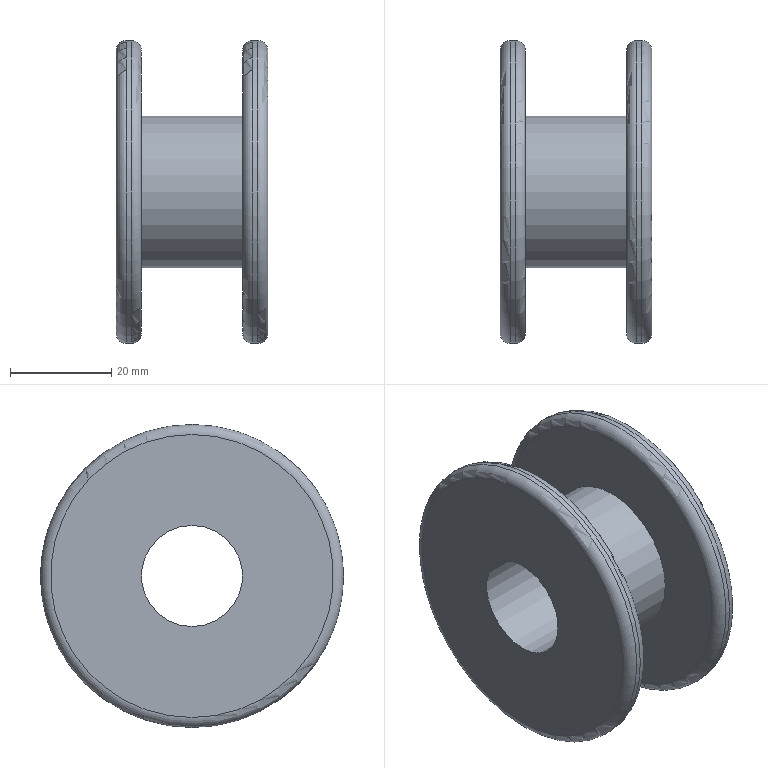Component | NX | 2 | 1 solid | 12 faces | box 30 x 60 x 60 mm | volume 32349 mm3 | cylinder 4 | plane 4 | torus 4 | commonest cylinder face diameters 60 x2 30 x1 20 x1
STEP:
#1=CARTESIAN_POINT('',(0.,0.,0.));
#2=DIRECTION('',(0.,0.,1.));
#3=DIRECTION('',(1.,0.,0.));
#4=AXIS2_PLACEMENT_3D('',#1,#2,#3);
#5=CARTESIAN_POINT('',(10.,0.,23.));
#6=VERTEX_POINT('',#5);
#7=CARTESIAN_POINT('',(10.,0.,38.));
#8=DIRECTION('',(1.,0.,0.));
#9=DIRECTION('',(0.,0.,-1.));
#10=AXIS2_PLACEMENT_3D('',#7,#8,#9);
#11=CIRCLE('',#10,15.);
#12=CARTESIAN_POINT('',(-15.,0.,38.));
#13=DIRECTION('',(1.,0.,0.));
#14=DIRECTION('',(0.,-1.,0.));
#15=AXIS2_PLACEMENT_3D('',#12,#13,#14);
#16=CYLINDRICAL_SURFACE('',#15,15.);
#17=CARTESIAN_POINT('',(1.571,25.));
#18=DIRECTION('',(1.,0.));
#19=VECTOR('',#18,1.);
#20=LINE('',#17,#19);
#21=(GEOMETRIC_REPRESENTATION_CONTEXT(2)PARAMETRIC_REPRESENTATION_CONTEXT()REPRESENTATION_CONTEXT('',''));
#22=DEFINITIONAL_REPRESENTATION('',(#20),#21);
#23=PCURVE('',#16,#22);
#24=CARTESIAN_POINT('',(10.,0.,38.));
#25=DIRECTION('',(-1.,0.,0.));
#26=DIRECTION('',(0.,0.,-1.));
#27=AXIS2_PLACEMENT_3D('',#24,#25,#26);
#28=PLANE('',#27);
#29=CARTESIAN_POINT('',(15.,0.));
#30=CARTESIAN_POINT('',(15.,-25.981));
#31=CARTESIAN_POINT('',(-7.5,-12.99));
#32=CARTESIAN_POINT('',(-30.,-0.));
#33=CARTESIAN_POINT('',(-7.5,12.99));
#34=CARTESIAN_POINT('',(15.,25.981));
#35=CARTESIAN_POINT('',(15.,0.));
#36=(BOUNDED_CURVE()B_SPLINE_CURVE(2,(#29,#30,#31,#32,#33,#34,#35),.UNSPECIFIED.,.T.,.F.)B_SPLINE_CURVE_WITH_KNOTS((1,2,2,2,2,1),(-2.094,0.,2.094,4.189,6.283,8.378),.UNSPECIFIED.)CURVE()GEOMETRIC_REPRESENTATION_ITEM()RATIONAL_B_SPLINE_CURVE((1.,0.5,1.,0.5,1.,0.5,1.))REPRESENTATION_ITEM(''));
#37=(GEOMETRIC_REPRESENTATION_CONTEXT(2)PARAMETRIC_REPRESENTATION_CONTEXT()REPRESENTATION_CONTEXT('',''));
#38=DEFINITIONAL_REPRESENTATION('',(#36),#37);
#39=PCURVE('',#28,#38);
#40=SURFACE_CURVE('',#11,(#23,#39),.PCURVE_S1.);
#41=EDGE_CURVE('',#6,#6,#40,.T.);
#42=ORIENTED_EDGE('',*,*,#41,.F.);
#43=CARTESIAN_POINT('',(-10.,-0.,23.));
#44=VERTEX_POINT('',#43);
#45=CARTESIAN_POINT('',(-10.,-0.,23.));
#46=CARTESIAN_POINT('',(10.,-0.,23.));
#47=B_SPLINE_CURVE_WITH_KNOTS('',1,(#45,#46),.UNSPECIFIED.,.F.,.F.,(2,2),(5.,25.),.PIECEWISE_BEZIER_KNOTS.);
#48=CARTESIAN_POINT('',(1.571,0.));
#49=DIRECTION('',(0.,1.));
#50=VECTOR('',#49,1.);
#51=LINE('',#48,#50);
#52=(GEOMETRIC_REPRESENTATION_CONTEXT(2)PARAMETRIC_REPRESENTATION_CONTEXT()REPRESENTATION_CONTEXT('',''));
#53=DEFINITIONAL_REPRESENTATION('',(#51),#52);
#54=PCURVE('',#16,#53);
#55=CARTESIAN_POINT('',(7.854,0.));
#56=DIRECTION('',(0.,1.));
#57=VECTOR('',#56,1.);
#58=LINE('',#55,#57);
#59=(GEOMETRIC_REPRESENTATION_CONTEXT(2)PARAMETRIC_REPRESENTATION_CONTEXT()REPRESENTATION_CONTEXT('',''));
#60=DEFINITIONAL_REPRESENTATION('',(#58),#59);
#61=PCURVE('',#16,#60);
#62=SEAM_CURVE('',#47,(#54,#61),.PCURVE_S1.);
#63=EDGE_CURVE('',#44,#6,#62,.T.);
#64=ORIENTED_EDGE('',*,*,#63,.F.);
#65=CARTESIAN_POINT('',(-10.,0.,53.));
#66=VERTEX_POINT('',#65);
#67=CARTESIAN_POINT('',(-10.,0.,38.));
#68=DIRECTION('',(-1.,0.,0.));
#69=DIRECTION('',(0.,0.,1.));
#70=AXIS2_PLACEMENT_3D('',#67,#68,#69);
#71=CIRCLE('',#70,15.);
#72=CARTESIAN_POINT('',(4.712,5.));
#73=DIRECTION('',(-1.,0.));
#74=VECTOR('',#73,1.);
#75=LINE('',#72,#74);
#76=(GEOMETRIC_REPRESENTATION_CONTEXT(2)PARAMETRIC_REPRESENTATION_CONTEXT()REPRESENTATION_CONTEXT('',''));
#77=DEFINITIONAL_REPRESENTATION('',(#75),#76);
#78=PCURVE('',#16,#77);
#79=CARTESIAN_POINT('',(-10.,0.,38.));
#80=DIRECTION('',(1.,0.,0.));
#81=DIRECTION('',(0.,0.,1.));
#82=AXIS2_PLACEMENT_3D('',#79,#80,#81);
#83=PLANE('',#82);
#84=CARTESIAN_POINT('',(15.,0.));
#85=CARTESIAN_POINT('',(15.,-25.981));
#86=CARTESIAN_POINT('',(-7.5,-12.99));
#87=CARTESIAN_POINT('',(-30.,-0.));
#88=CARTESIAN_POINT('',(-7.5,12.99));
#89=CARTESIAN_POINT('',(15.,25.981));
#90=CARTESIAN_POINT('',(15.,0.));
#91=(BOUNDED_CURVE()B_SPLINE_CURVE(2,(#84,#85,#86,#87,#88,#89,#90),.UNSPECIFIED.,.T.,.F.)B_SPLINE_CURVE_WITH_KNOTS((1,2,2,2,2,1),(-2.094,0.,2.094,4.189,6.283,8.378),.UNSPECIFIED.)CURVE()GEOMETRIC_REPRESENTATION_ITEM()RATIONAL_B_SPLINE_CURVE((1.,0.5,1.,0.5,1.,0.5,1.))REPRESENTATION_ITEM(''));
#92=(GEOMETRIC_REPRESENTATION_CONTEXT(2)PARAMETRIC_REPRESENTATION_CONTEXT()REPRESENTATION_CONTEXT('',''));
#93=DEFINITIONAL_REPRESENTATION('',(#91),#92);
#94=PCURVE('',#83,#93);
#95=SURFACE_CURVE('',#71,(#78,#94),.PCURVE_S1.);
#96=EDGE_CURVE('',#66,#44,#95,.T.);
#97=ORIENTED_EDGE('',*,*,#96,.F.);
#98=CARTESIAN_POINT('',(-10.,0.,38.));
#99=DIRECTION('',(-1.,0.,0.));
#100=DIRECTION('',(0.,0.,1.));
#101=AXIS2_PLACEMENT_3D('',#98,#99,#100);
#102=CIRCLE('',#101,15.);
#103=CARTESIAN_POINT('',(10.996,5.));
#104=DIRECTION('',(-1.,0.));
#105=VECTOR('',#104,1.);
#106=LINE('',#103,#105);
#107=(GEOMETRIC_REPRESENTATION_CONTEXT(2)PARAMETRIC_REPRESENTATION_CONTEXT()REPRESENTATION_CONTEXT('',''));
#108=DEFINITIONAL_REPRESENTATION('',(#106),#107);
#109=PCURVE('',#16,#108);
#110=CARTESIAN_POINT('',(15.,0.));
#111=CARTESIAN_POINT('',(15.,-25.981));
#112=CARTESIAN_POINT('',(-7.5,-12.99));
#113=CARTESIAN_POINT('',(-30.,-0.));
#114=CARTESIAN_POINT('',(-7.5,12.99));
#115=CARTESIAN_POINT('',(15.,25.981));
#116=CARTESIAN_POINT('',(15.,0.));
#117=(BOUNDED_CURVE()B_SPLINE_CURVE(2,(#110,#111,#112,#113,#114,#115,#116),.UNSPECIFIED.,.T.,.F.)B_SPLINE_CURVE_WITH_KNOTS((1,2,2,2,2,1),(-2.094,0.,2.094,4.189,6.283,8.378),.UNSPECIFIED.)CURVE()GEOMETRIC_REPRESENTATION_ITEM()RATIONAL_B_SPLINE_CURVE((1.,0.5,1.,0.5,1.,0.5,1.))REPRESENTATION_ITEM(''));
#118=(GEOMETRIC_REPRESENTATION_CONTEXT(2)PARAMETRIC_REPRESENTATION_CONTEXT()REPRESENTATION_CONTEXT('',''));
#119=DEFINITIONAL_REPRESENTATION('',(#117),#118);
#120=PCURVE('',#83,#119);
#121=SURFACE_CURVE('',#102,(#109,#120),.PCURVE_S1.);
#122=EDGE_CURVE('',#44,#66,#121,.T.);
#123=ORIENTED_EDGE('',*,*,#122,.F.);
#124=ORIENTED_EDGE('',*,*,#63,.T.);
#125=EDGE_LOOP('',(#42,#64,#97,#123,#124));
#126=FACE_BOUND('',#125,.T.);
#127=ADVANCED_FACE('',(#126),#16,.T.);
#128=CARTESIAN_POINT('',(-10.,0.,66.));
#129=VERTEX_POINT('',#128);
#130=CARTESIAN_POINT('',(-10.,0.,38.));
#131=DIRECTION('',(1.,0.,0.));
#132=DIRECTION('',(0.,0.,1.));
#133=AXIS2_PLACEMENT_3D('',#130,#131,#132);
#134=CIRCLE('',#133,28.);
#135=CARTESIAN_POINT('',(0.,0.));
#136=DIRECTION('',(1.,0.));
#137=AXIS2_PLACEMENT_2D('',#135,#136);
#138=CIRCLE('',#137,28.);
#139=(GEOMETRIC_REPRESENTATION_CONTEXT(2)PARAMETRIC_REPRESENTATION_CONTEXT()REPRESENTATION_CONTEXT('',''));
#140=DEFINITIONAL_REPRESENTATION('',(#138),#139);
#141=PCURVE('',#83,#140);
#142=CARTESIAN_POINT('',(-12.,0.,38.));
#143=DIRECTION('',(1.,0.,0.));
#144=DIRECTION('',(0.,0.,1.));
#145=AXIS2_PLACEMENT_3D('',#142,#143,#144);
#146=TOROIDAL_SURFACE('',#145,28.,2.);
#147=CARTESIAN_POINT('',(0.,7.854));
#148=DIRECTION('',(1.,0.));
#149=VECTOR('',#148,1.);
#150=LINE('',#147,#149);
#151=(GEOMETRIC_REPRESENTATION_CONTEXT(2)PARAMETRIC_REPRESENTATION_CONTEXT()REPRESENTATION_CONTEXT('',''));
#152=DEFINITIONAL_REPRESENTATION('',(#150),#151);
#153=PCURVE('',#146,#152);
#154=SURFACE_CURVE('',#134,(#141,#153),.PCURVE_S1.);
#155=EDGE_CURVE('',#129,#129,#154,.T.);
#156=ORIENTED_EDGE('',*,*,#155,.T.);
#157=EDGE_LOOP('',(#156));
#158=FACE_BOUND('',#157,.T.);
#159=ORIENTED_EDGE('',*,*,#96,.T.);
#160=ORIENTED_EDGE('',*,*,#122,.T.);
#161=EDGE_LOOP('',(#159,#160));
#162=FACE_BOUND('',#161,.T.);
#163=ADVANCED_FACE('',(#158,#162),#83,.T.);
#164=CARTESIAN_POINT('',(-12.,0.,68.));
#165=VERTEX_POINT('',#164);
#166=CARTESIAN_POINT('',(-12.,0.,38.));
#167=DIRECTION('',(-1.,0.,0.));
#168=DIRECTION('',(0.,0.,1.));
#169=AXIS2_PLACEMENT_3D('',#166,#167,#168);
#170=CIRCLE('',#169,30.);
#171=CARTESIAN_POINT('',(-15.,0.,38.));
#172=DIRECTION('',(1.,0.,0.));
#173=DIRECTION('',(0.,-1.,0.));
#174=AXIS2_PLACEMENT_3D('',#171,#172,#173);
#175=CYLINDRICAL_SURFACE('',#174,30.);
#176=CARTESIAN_POINT('',(10.996,3.));
#177=DIRECTION('',(-1.,0.));
#178=VECTOR('',#177,1.);
#179=LINE('',#176,#178);
#180=(GEOMETRIC_REPRESENTATION_CONTEXT(2)PARAMETRIC_REPRESENTATION_CONTEXT()REPRESENTATION_CONTEXT('',''));
#181=DEFINITIONAL_REPRESENTATION('',(#179),#180);
#182=PCURVE('',#175,#181);
#183=CARTESIAN_POINT('',(6.283,6.283));
#184=DIRECTION('',(-1.,0.));
#185=VECTOR('',#184,1.);
#186=LINE('',#183,#185);
#187=(GEOMETRIC_REPRESENTATION_CONTEXT(2)PARAMETRIC_REPRESENTATION_CONTEXT()REPRESENTATION_CONTEXT('',''));
#188=DEFINITIONAL_REPRESENTATION('',(#186),#187);
#189=PCURVE('',#146,#188);
#190=SURFACE_CURVE('',#170,(#182,#189),.PCURVE_S1.);
#191=EDGE_CURVE('',#165,#165,#190,.T.);
#192=ORIENTED_EDGE('',*,*,#191,.T.);
#193=CARTESIAN_POINT('',(-13.,0.,68.));
#194=VERTEX_POINT('',#193);
#195=CARTESIAN_POINT('',(-13.,0.,68.));
#196=CARTESIAN_POINT('',(-12.,0.,68.));
#197=B_SPLINE_CURVE_WITH_KNOTS('',1,(#195,#196),.UNSPECIFIED.,.F.,.F.,(2,2),(2.,3.),.PIECEWISE_BEZIER_KNOTS.);
#198=CARTESIAN_POINT('',(4.712,0.));
#199=DIRECTION('',(0.,1.));
#200=VECTOR('',#199,1.);
#201=LINE('',#198,#200);
#202=(GEOMETRIC_REPRESENTATION_CONTEXT(2)PARAMETRIC_REPRESENTATION_CONTEXT()REPRESENTATION_CONTEXT('',''));
#203=DEFINITIONAL_REPRESENTATION('',(#201),#202);
#204=PCURVE('',#175,#203);
#205=CARTESIAN_POINT('',(10.996,0.));
#206=DIRECTION('',(0.,1.));
#207=VECTOR('',#206,1.);
#208=LINE('',#205,#207);
#209=(GEOMETRIC_REPRESENTATION_CONTEXT(2)PARAMETRIC_REPRESENTATION_CONTEXT()REPRESENTATION_CONTEXT('',''));
#210=DEFINITIONAL_REPRESENTATION('',(#208),#209);
#211=PCURVE('',#175,#210);
#212=SEAM_CURVE('',#197,(#204,#211),.PCURVE_S1.);
#213=EDGE_CURVE('',#194,#165,#212,.T.);
#214=ORIENTED_EDGE('',*,*,#213,.F.);
#215=CARTESIAN_POINT('',(-13.,0.,8.));
#216=VERTEX_POINT('',#215);
#217=CARTESIAN_POINT('',(-13.,0.,38.));
#218=DIRECTION('',(1.,0.,0.));
#219=DIRECTION('',(0.,0.,-1.));
#220=AXIS2_PLACEMENT_3D('',#217,#218,#219);
#221=CIRCLE('',#220,30.);
#222=CARTESIAN_POINT('',(1.571,2.));
#223=DIRECTION('',(1.,0.));
#224=VECTOR('',#223,1.);
#225=LINE('',#222,#224);
#226=(GEOMETRIC_REPRESENTATION_CONTEXT(2)PARAMETRIC_REPRESENTATION_CONTEXT()REPRESENTATION_CONTEXT('',''));
#227=DEFINITIONAL_REPRESENTATION('',(#225),#226);
#228=PCURVE('',#175,#227);
#229=CARTESIAN_POINT('',(-13.,0.,38.));
#230=DIRECTION('',(-1.,0.,0.));
#231=DIRECTION('',(0.,0.,-1.));
#232=AXIS2_PLACEMENT_3D('',#229,#230,#231);
#233=TOROIDAL_SURFACE('',#232,28.,2.);
#234=CARTESIAN_POINT('',(6.283,6.283));
#235=DIRECTION('',(-1.,0.));
#236=VECTOR('',#235,1.);
#237=LINE('',#234,#236);
#238=(GEOMETRIC_REPRESENTATION_CONTEXT(2)PARAMETRIC_REPRESENTATION_CONTEXT()REPRESENTATION_CONTEXT('',''));
#239=DEFINITIONAL_REPRESENTATION('',(#237),#238);
#240=PCURVE('',#233,#239);
#241=SURFACE_CURVE('',#221,(#228,#240),.PCURVE_S1.);
#242=EDGE_CURVE('',#194,#216,#241,.T.);
#243=ORIENTED_EDGE('',*,*,#242,.T.);
#244=CARTESIAN_POINT('',(-13.,0.,38.));
#245=DIRECTION('',(1.,0.,0.));
#246=DIRECTION('',(0.,0.,-1.));
#247=AXIS2_PLACEMENT_3D('',#244,#245,#246);
#248=CIRCLE('',#247,30.);
#249=CARTESIAN_POINT('',(7.854,2.));
#250=DIRECTION('',(1.,0.));
#251=VECTOR('',#250,1.);
#252=LINE('',#249,#251);
#253=(GEOMETRIC_REPRESENTATION_CONTEXT(2)PARAMETRIC_REPRESENTATION_CONTEXT()REPRESENTATION_CONTEXT('',''));
#254=DEFINITIONAL_REPRESENTATION('',(#252),#253);
#255=PCURVE('',#175,#254);
#256=CARTESIAN_POINT('',(6.283,6.283));
#257=DIRECTION('',(-1.,0.));
#258=VECTOR('',#257,1.);
#259=LINE('',#256,#258);
#260=(GEOMETRIC_REPRESENTATION_CONTEXT(2)PARAMETRIC_REPRESENTATION_CONTEXT()REPRESENTATION_CONTEXT('',''));
#261=DEFINITIONAL_REPRESENTATION('',(#259),#260);
#262=PCURVE('',#233,#261);
#263=SURFACE_CURVE('',#248,(#255,#262),.PCURVE_S1.);
#264=EDGE_CURVE('',#216,#194,#263,.T.);
#265=ORIENTED_EDGE('',*,*,#264,.T.);
#266=ORIENTED_EDGE('',*,*,#213,.T.);
#267=EDGE_LOOP('',(#192,#214,#243,#265,#266));
#268=FACE_BOUND('',#267,.T.);
#269=ADVANCED_FACE('',(#268),#175,.T.);
#270=CARTESIAN_POINT('',(-15.,0.,10.));
#271=VERTEX_POINT('',#270);
#272=CARTESIAN_POINT('',(-15.,0.,38.));
#273=DIRECTION('',(-1.,0.,0.));
#274=DIRECTION('',(0.,0.,-1.));
#275=AXIS2_PLACEMENT_3D('',#272,#273,#274);
#276=CIRCLE('',#275,28.);
#277=CARTESIAN_POINT('',(-15.,0.,38.));
#278=DIRECTION('',(-1.,0.,0.));
#279=DIRECTION('',(0.,0.,-1.));
#280=AXIS2_PLACEMENT_3D('',#277,#278,#279);
#281=PLANE('',#280);
#282=CARTESIAN_POINT('',(0.,0.));
#283=DIRECTION('',(1.,0.));
#284=AXIS2_PLACEMENT_2D('',#282,#283);
#285=CIRCLE('',#284,28.);
#286=(GEOMETRIC_REPRESENTATION_CONTEXT(2)PARAMETRIC_REPRESENTATION_CONTEXT()REPRESENTATION_CONTEXT('',''));
#287=DEFINITIONAL_REPRESENTATION('',(#285),#286);
#288=PCURVE('',#281,#287);
#289=CARTESIAN_POINT('',(0.,7.854));
#290=DIRECTION('',(1.,0.));
#291=VECTOR('',#290,1.);
#292=LINE('',#289,#291);
#293=(GEOMETRIC_REPRESENTATION_CONTEXT(2)PARAMETRIC_REPRESENTATION_CONTEXT()REPRESENTATION_CONTEXT('',''));
#294=DEFINITIONAL_REPRESENTATION('',(#292),#293);
#295=PCURVE('',#233,#294);
#296=SURFACE_CURVE('',#276,(#288,#295),.PCURVE_S1.);
#297=EDGE_CURVE('',#271,#271,#296,.T.);
#298=ORIENTED_EDGE('',*,*,#297,.T.);
#299=EDGE_LOOP('',(#298));
#300=FACE_BOUND('',#299,.T.);
#301=CARTESIAN_POINT('',(-15.,0.,48.));
#302=VERTEX_POINT('',#301);
#303=CARTESIAN_POINT('',(-15.,0.,38.));
#304=DIRECTION('',(1.,0.,0.));
#305=DIRECTION('',(0.,0.,1.));
#306=AXIS2_PLACEMENT_3D('',#303,#304,#305);
#307=CIRCLE('',#306,10.);
#308=CARTESIAN_POINT('',(-10.,0.));
#309=CARTESIAN_POINT('',(-10.,17.321));
#310=CARTESIAN_POINT('',(5.,8.66));
#311=CARTESIAN_POINT('',(20.,0.));
#312=CARTESIAN_POINT('',(5.,-8.66));
#313=CARTESIAN_POINT('',(-10.,-17.321));
#314=CARTESIAN_POINT('',(-10.,0.));
#315=(BOUNDED_CURVE()B_SPLINE_CURVE(2,(#308,#309,#310,#311,#312,#313,#314),.UNSPECIFIED.,.T.,.F.)B_SPLINE_CURVE_WITH_KNOTS((1,2,2,2,2,1),(-2.094,0.,2.094,4.189,6.283,8.378),.UNSPECIFIED.)CURVE()GEOMETRIC_REPRESENTATION_ITEM()RATIONAL_B_SPLINE_CURVE((1.,0.5,1.,0.5,1.,0.5,1.))REPRESENTATION_ITEM(''));
#316=(GEOMETRIC_REPRESENTATION_CONTEXT(2)PARAMETRIC_REPRESENTATION_CONTEXT()REPRESENTATION_CONTEXT('',''));
#317=DEFINITIONAL_REPRESENTATION('',(#315),#316);
#318=PCURVE('',#281,#317);
#319=CARTESIAN_POINT('',(-15.,0.,38.));
#320=DIRECTION('',(1.,0.,0.));
#321=DIRECTION('',(0.,0.,1.));
#322=AXIS2_PLACEMENT_3D('',#319,#320,#321);
#323=CYLINDRICAL_SURFACE('',#322,10.);
#324=CARTESIAN_POINT('',(0.,0.));
#325=DIRECTION('',(1.,0.));
#326=VECTOR('',#325,1.);
#327=LINE('',#324,#326);
#328=(GEOMETRIC_REPRESENTATION_CONTEXT(2)PARAMETRIC_REPRESENTATION_CONTEXT()REPRESENTATION_CONTEXT('',''));
#329=DEFINITIONAL_REPRESENTATION('',(#327),#328);
#330=PCURVE('',#323,#329);
#331=SURFACE_CURVE('',#307,(#318,#330),.PCURVE_S1.);
#332=EDGE_CURVE('',#302,#302,#331,.T.);
#333=ORIENTED_EDGE('',*,*,#332,.T.);
#334=EDGE_LOOP('',(#333));
#335=FACE_BOUND('',#334,.T.);
#336=ADVANCED_FACE('',(#300,#335),#281,.T.);
#337=CARTESIAN_POINT('',(10.,0.,10.));
#338=VERTEX_POINT('',#337);
#339=CARTESIAN_POINT('',(10.,0.,38.));
#340=DIRECTION('',(-1.,0.,0.));
#341=DIRECTION('',(0.,0.,-1.));
#342=AXIS2_PLACEMENT_3D('',#339,#340,#341);
#343=CIRCLE('',#342,28.);
#344=CARTESIAN_POINT('',(0.,0.));
#345=DIRECTION('',(1.,0.));
#346=AXIS2_PLACEMENT_2D('',#344,#345);
#347=CIRCLE('',#346,28.);
#348=(GEOMETRIC_REPRESENTATION_CONTEXT(2)PARAMETRIC_REPRESENTATION_CONTEXT()REPRESENTATION_CONTEXT('',''));
#349=DEFINITIONAL_REPRESENTATION('',(#347),#348);
#350=PCURVE('',#28,#349);
#351=CARTESIAN_POINT('',(12.,0.,38.));
#352=DIRECTION('',(-1.,0.,0.));
#353=DIRECTION('',(0.,0.,-1.));
#354=AXIS2_PLACEMENT_3D('',#351,#352,#353);
#355=TOROIDAL_SURFACE('',#354,28.,2.);
#356=CARTESIAN_POINT('',(0.,7.854));
#357=DIRECTION('',(1.,0.));
#358=VECTOR('',#357,1.);
#359=LINE('',#356,#358);
#360=(GEOMETRIC_REPRESENTATION_CONTEXT(2)PARAMETRIC_REPRESENTATION_CONTEXT()REPRESENTATION_CONTEXT('',''));
#361=DEFINITIONAL_REPRESENTATION('',(#359),#360);
#362=PCURVE('',#355,#361);
#363=SURFACE_CURVE('',#343,(#350,#362),.PCURVE_S1.);
#364=EDGE_CURVE('',#338,#338,#363,.T.);
#365=ORIENTED_EDGE('',*,*,#364,.T.);
#366=EDGE_LOOP('',(#365));
#367=FACE_BOUND('',#366,.T.);
#368=ORIENTED_EDGE('',*,*,#41,.T.);
#369=EDGE_LOOP('',(#368));
#370=FACE_BOUND('',#369,.T.);
#371=ADVANCED_FACE('',(#367,#370),#28,.T.);
#372=CARTESIAN_POINT('',(13.,0.,68.));
#373=VERTEX_POINT('',#372);
#374=CARTESIAN_POINT('',(13.,0.,38.));
#375=DIRECTION('',(-1.,0.,0.));
#376=DIRECTION('',(0.,0.,1.));
#377=AXIS2_PLACEMENT_3D('',#374,#375,#376);
#378=CIRCLE('',#377,30.);
#379=CARTESIAN_POINT('',(15.,0.,38.));
#380=DIRECTION('',(-1.,0.,0.));
#381=DIRECTION('',(0.,-1.,0.));
#382=AXIS2_PLACEMENT_3D('',#379,#380,#381);
#383=CYLINDRICAL_SURFACE('',#382,30.);
#384=CARTESIAN_POINT('',(1.571,2.));
#385=DIRECTION('',(1.,0.));
#386=VECTOR('',#385,1.);
#387=LINE('',#384,#386);
#388=(GEOMETRIC_REPRESENTATION_CONTEXT(2)PARAMETRIC_REPRESENTATION_CONTEXT()REPRESENTATION_CONTEXT('',''));
#389=DEFINITIONAL_REPRESENTATION('',(#387),#388);
#390=PCURVE('',#383,#389);
#391=CARTESIAN_POINT('',(13.,0.,38.));
#392=DIRECTION('',(1.,0.,0.));
#393=DIRECTION('',(0.,0.,1.));
#394=AXIS2_PLACEMENT_3D('',#391,#392,#393);
#395=TOROIDAL_SURFACE('',#394,28.,2.);
#396=CARTESIAN_POINT('',(6.283,6.283));
#397=DIRECTION('',(-1.,0.));
#398=VECTOR('',#397,1.);
#399=LINE('',#396,#398);
#400=(GEOMETRIC_REPRESENTATION_CONTEXT(2)PARAMETRIC_REPRESENTATION_CONTEXT()REPRESENTATION_CONTEXT('',''));
#401=DEFINITIONAL_REPRESENTATION('',(#399),#400);
#402=PCURVE('',#395,#401);
#403=SURFACE_CURVE('',#378,(#390,#402),.PCURVE_S1.);
#404=EDGE_CURVE('',#373,#373,#403,.T.);
#405=ORIENTED_EDGE('',*,*,#404,.T.);
#406=CARTESIAN_POINT('',(12.,-0.,68.));
#407=VERTEX_POINT('',#406);
#408=CARTESIAN_POINT('',(13.,-0.,68.));
#409=CARTESIAN_POINT('',(12.,-0.,68.));
#410=B_SPLINE_CURVE_WITH_KNOTS('',1,(#408,#409),.UNSPECIFIED.,.F.,.F.,(2,2),(2.,3.),.PIECEWISE_BEZIER_KNOTS.);
#411=CARTESIAN_POINT('',(7.854,0.));
#412=DIRECTION('',(0.,1.));
#413=VECTOR('',#412,1.);
#414=LINE('',#411,#413);
#415=(GEOMETRIC_REPRESENTATION_CONTEXT(2)PARAMETRIC_REPRESENTATION_CONTEXT()REPRESENTATION_CONTEXT('',''));
#416=DEFINITIONAL_REPRESENTATION('',(#414),#415);
#417=PCURVE('',#383,#416);
#418=CARTESIAN_POINT('',(1.571,0.));
#419=DIRECTION('',(0.,1.));
#420=VECTOR('',#419,1.);
#421=LINE('',#418,#420);
#422=(GEOMETRIC_REPRESENTATION_CONTEXT(2)PARAMETRIC_REPRESENTATION_CONTEXT()REPRESENTATION_CONTEXT('',''));
#423=DEFINITIONAL_REPRESENTATION('',(#421),#422);
#424=PCURVE('',#383,#423);
#425=SEAM_CURVE('',#410,(#417,#424),.PCURVE_S1.);
#426=EDGE_CURVE('',#373,#407,#425,.T.);
#427=ORIENTED_EDGE('',*,*,#426,.T.);
#428=CARTESIAN_POINT('',(12.,0.,8.));
#429=VERTEX_POINT('',#428);
#430=CARTESIAN_POINT('',(12.,0.,38.));
#431=DIRECTION('',(1.,0.,0.));
#432=DIRECTION('',(0.,0.,-1.));
#433=AXIS2_PLACEMENT_3D('',#430,#431,#432);
#434=CIRCLE('',#433,30.);
#435=CARTESIAN_POINT('',(10.996,3.));
#436=DIRECTION('',(-1.,0.));
#437=VECTOR('',#436,1.);
#438=LINE('',#435,#437);
#439=(GEOMETRIC_REPRESENTATION_CONTEXT(2)PARAMETRIC_REPRESENTATION_CONTEXT()REPRESENTATION_CONTEXT('',''));
#440=DEFINITIONAL_REPRESENTATION('',(#438),#439);
#441=PCURVE('',#383,#440);
#442=CARTESIAN_POINT('',(6.283,6.283));
#443=DIRECTION('',(-1.,0.));
#444=VECTOR('',#443,1.);
#445=LINE('',#442,#444);
#446=(GEOMETRIC_REPRESENTATION_CONTEXT(2)PARAMETRIC_REPRESENTATION_CONTEXT()REPRESENTATION_CONTEXT('',''));
#447=DEFINITIONAL_REPRESENTATION('',(#445),#446);
#448=PCURVE('',#355,#447);
#449=SURFACE_CURVE('',#434,(#441,#448),.PCURVE_S1.);
#450=EDGE_CURVE('',#407,#429,#449,.T.);
#451=ORIENTED_EDGE('',*,*,#450,.T.);
#452=CARTESIAN_POINT('',(12.,0.,38.));
#453=DIRECTION('',(1.,0.,0.));
#454=DIRECTION('',(0.,0.,-1.));
#455=AXIS2_PLACEMENT_3D('',#452,#453,#454);
#456=CIRCLE('',#455,30.);
#457=CARTESIAN_POINT('',(4.712,3.));
#458=DIRECTION('',(-1.,0.));
#459=VECTOR('',#458,1.);
#460=LINE('',#457,#459);
#461=(GEOMETRIC_REPRESENTATION_CONTEXT(2)PARAMETRIC_REPRESENTATION_CONTEXT()REPRESENTATION_CONTEXT('',''));
#462=DEFINITIONAL_REPRESENTATION('',(#460),#461);
#463=PCURVE('',#383,#462);
#464=CARTESIAN_POINT('',(6.283,6.283));
#465=DIRECTION('',(-1.,0.));
#466=VECTOR('',#465,1.);
#467=LINE('',#464,#466);
#468=(GEOMETRIC_REPRESENTATION_CONTEXT(2)PARAMETRIC_REPRESENTATION_CONTEXT()REPRESENTATION_CONTEXT('',''));
#469=DEFINITIONAL_REPRESENTATION('',(#467),#468);
#470=PCURVE('',#355,#469);
#471=SURFACE_CURVE('',#456,(#463,#470),.PCURVE_S1.);
#472=EDGE_CURVE('',#429,#407,#471,.T.);
#473=ORIENTED_EDGE('',*,*,#472,.T.);
#474=ORIENTED_EDGE('',*,*,#426,.F.);
#475=EDGE_LOOP('',(#405,#427,#451,#473,#474));
#476=FACE_BOUND('',#475,.T.);
#477=ADVANCED_FACE('',(#476),#383,.T.);
#478=CARTESIAN_POINT('',(15.,0.,66.));
#479=VERTEX_POINT('',#478);
#480=CARTESIAN_POINT('',(15.,0.,38.));
#481=DIRECTION('',(1.,0.,0.));
#482=DIRECTION('',(0.,0.,1.));
#483=AXIS2_PLACEMENT_3D('',#480,#481,#482);
#484=CIRCLE('',#483,28.);
#485=CARTESIAN_POINT('',(15.,0.,38.));
#486=DIRECTION('',(1.,0.,0.));
#487=DIRECTION('',(0.,0.,1.));
#488=AXIS2_PLACEMENT_3D('',#485,#486,#487);
#489=PLANE('',#488);
#490=CARTESIAN_POINT('',(0.,0.));
#491=DIRECTION('',(1.,0.));
#492=AXIS2_PLACEMENT_2D('',#490,#491);
#493=CIRCLE('',#492,28.);
#494=(GEOMETRIC_REPRESENTATION_CONTEXT(2)PARAMETRIC_REPRESENTATION_CONTEXT()REPRESENTATION_CONTEXT('',''));
#495=DEFINITIONAL_REPRESENTATION('',(#493),#494);
#496=PCURVE('',#489,#495);
#497=CARTESIAN_POINT('',(0.,7.854));
#498=DIRECTION('',(1.,0.));
#499=VECTOR('',#498,1.);
#500=LINE('',#497,#499);
#501=(GEOMETRIC_REPRESENTATION_CONTEXT(2)PARAMETRIC_REPRESENTATION_CONTEXT()REPRESENTATION_CONTEXT('',''));
#502=DEFINITIONAL_REPRESENTATION('',(#500),#501);
#503=PCURVE('',#395,#502);
#504=SURFACE_CURVE('',#484,(#496,#503),.PCURVE_S1.);
#505=EDGE_CURVE('',#479,#479,#504,.T.);
#506=ORIENTED_EDGE('',*,*,#505,.T.);
#507=EDGE_LOOP('',(#506));
#508=FACE_BOUND('',#507,.T.);
#509=CARTESIAN_POINT('',(15.,0.,48.));
#510=VERTEX_POINT('',#509);
#511=CARTESIAN_POINT('',(15.,0.,38.));
#512=DIRECTION('',(1.,0.,0.));
#513=DIRECTION('',(0.,0.,1.));
#514=AXIS2_PLACEMENT_3D('',#511,#512,#513);
#515=CIRCLE('',#514,10.);
#516=CARTESIAN_POINT('',(0.,0.));
#517=DIRECTION('',(1.,0.));
#518=AXIS2_PLACEMENT_2D('',#516,#517);
#519=CIRCLE('',#518,10.);
#520=(GEOMETRIC_REPRESENTATION_CONTEXT(2)PARAMETRIC_REPRESENTATION_CONTEXT()REPRESENTATION_CONTEXT('',''));
#521=DEFINITIONAL_REPRESENTATION('',(#519),#520);
#522=PCURVE('',#489,#521);
#523=CARTESIAN_POINT('',(0.,30.));
#524=DIRECTION('',(1.,0.));
#525=VECTOR('',#524,1.);
#526=LINE('',#523,#525);
#527=(GEOMETRIC_REPRESENTATION_CONTEXT(2)PARAMETRIC_REPRESENTATION_CONTEXT()REPRESENTATION_CONTEXT('',''));
#528=DEFINITIONAL_REPRESENTATION('',(#526),#527);
#529=PCURVE('',#323,#528);
#530=SURFACE_CURVE('',#515,(#522,#529),.PCURVE_S1.);
#531=EDGE_CURVE('',#510,#510,#530,.T.);
#532=ORIENTED_EDGE('',*,*,#531,.F.);
#533=EDGE_LOOP('',(#532));
#534=FACE_BOUND('',#533,.T.);
#535=ADVANCED_FACE('',(#508,#534),#489,.T.);
#536=ORIENTED_EDGE('',*,*,#531,.F.);
#537=CARTESIAN_POINT('',(-15.,0.,48.));
#538=CARTESIAN_POINT('',(15.,0.,48.));
#539=B_SPLINE_CURVE_WITH_KNOTS('',1,(#537,#538),.UNSPECIFIED.,.F.,.F.,(2,2),(0.,30.),.PIECEWISE_BEZIER_KNOTS.);
#540=CARTESIAN_POINT('',(0.,0.));
#541=DIRECTION('',(0.,1.));
#542=VECTOR('',#541,1.);
#543=LINE('',#540,#542);
#544=(GEOMETRIC_REPRESENTATION_CONTEXT(2)PARAMETRIC_REPRESENTATION_CONTEXT()REPRESENTATION_CONTEXT('',''));
#545=DEFINITIONAL_REPRESENTATION('',(#543),#544);
#546=PCURVE('',#323,#545);
#547=CARTESIAN_POINT('',(6.283,0.));
#548=DIRECTION('',(0.,1.));
#549=VECTOR('',#548,1.);
#550=LINE('',#547,#549);
#551=(GEOMETRIC_REPRESENTATION_CONTEXT(2)PARAMETRIC_REPRESENTATION_CONTEXT()REPRESENTATION_CONTEXT('',''));
#552=DEFINITIONAL_REPRESENTATION('',(#550),#551);
#553=PCURVE('',#323,#552);
#554=SEAM_CURVE('',#539,(#546,#553),.PCURVE_S1.);
#555=EDGE_CURVE('',#302,#510,#554,.T.);
#556=ORIENTED_EDGE('',*,*,#555,.F.);
#557=ORIENTED_EDGE('',*,*,#332,.T.);
#558=ORIENTED_EDGE('',*,*,#555,.T.);
#559=EDGE_LOOP('',(#536,#556,#557,#558));
#560=FACE_BOUND('',#559,.F.);
#561=ADVANCED_FACE('',(#560),#323,.F.);
#562=ORIENTED_EDGE('',*,*,#505,.F.);
#563=CARTESIAN_POINT('',(13.,0.,68.));
#564=CARTESIAN_POINT('',(13.535,0.,68.));
#565=CARTESIAN_POINT('',(14.055,0.,67.83));
#566=CARTESIAN_POINT('',(14.504,0.,67.504));
#567=CARTESIAN_POINT('',(14.83,0.,67.055));
#568=CARTESIAN_POINT('',(15.,0.,66.535));
#569=CARTESIAN_POINT('',(15.,0.,66.));
#570=(BOUNDED_CURVE()B_SPLINE_CURVE(6,(#563,#564,#565,#566,#567,#568,#569),.UNSPECIFIED.,.F.,.F.)B_SPLINE_CURVE_WITH_KNOTS((7,7),(0.,1.571),.PIECEWISE_BEZIER_KNOTS.)CURVE()GEOMETRIC_REPRESENTATION_ITEM()RATIONAL_B_SPLINE_CURVE((1.031,1.01,0.9979,0.994,0.9979,1.01,1.031))REPRESENTATION_ITEM(''));
#571=CARTESIAN_POINT('',(0.,6.283));
#572=DIRECTION('',(0.,1.));
#573=VECTOR('',#572,1.);
#574=LINE('',#571,#573);
#575=(GEOMETRIC_REPRESENTATION_CONTEXT(2)PARAMETRIC_REPRESENTATION_CONTEXT()REPRESENTATION_CONTEXT('',''));
#576=DEFINITIONAL_REPRESENTATION('',(#574),#575);
#577=PCURVE('',#395,#576);
#578=CARTESIAN_POINT('',(6.283,6.283));
#579=DIRECTION('',(0.,1.));
#580=VECTOR('',#579,1.);
#581=LINE('',#578,#580);
#582=(GEOMETRIC_REPRESENTATION_CONTEXT(2)PARAMETRIC_REPRESENTATION_CONTEXT()REPRESENTATION_CONTEXT('',''));
#583=DEFINITIONAL_REPRESENTATION('',(#581),#582);
#584=PCURVE('',#395,#583);
#585=SEAM_CURVE('',#570,(#577,#584),.PCURVE_S1.);
#586=EDGE_CURVE('',#373,#479,#585,.T.);
#587=ORIENTED_EDGE('',*,*,#586,.F.);
#588=ORIENTED_EDGE('',*,*,#404,.F.);
#589=ORIENTED_EDGE('',*,*,#586,.T.);
#590=EDGE_LOOP('',(#562,#587,#588,#589));
#591=FACE_BOUND('',#590,.T.);
#592=ADVANCED_FACE('',(#591),#395,.T.);
#593=ORIENTED_EDGE('',*,*,#364,.F.);
#594=CARTESIAN_POINT('',(12.,0.,8.));
#595=CARTESIAN_POINT('',(11.465,0.,8.));
#596=CARTESIAN_POINT('',(10.945,0.,8.17));
#597=CARTESIAN_POINT('',(10.496,0.,8.496));
#598=CARTESIAN_POINT('',(10.17,0.,8.945));
#599=CARTESIAN_POINT('',(10.,0.,9.465));
#600=CARTESIAN_POINT('',(10.,0.,10.));
#601=(BOUNDED_CURVE()B_SPLINE_CURVE(6,(#594,#595,#596,#597,#598,#599,#600),.UNSPECIFIED.,.F.,.F.)B_SPLINE_CURVE_WITH_KNOTS((7,7),(0.,1.571),.PIECEWISE_BEZIER_KNOTS.)CURVE()GEOMETRIC_REPRESENTATION_ITEM()RATIONAL_B_SPLINE_CURVE((1.031,1.01,0.9979,0.994,0.9979,1.01,1.031))REPRESENTATION_ITEM(''));
#602=CARTESIAN_POINT('',(0.,6.283));
#603=DIRECTION('',(0.,1.));
#604=VECTOR('',#603,1.);
#605=LINE('',#602,#604);
#606=(GEOMETRIC_REPRESENTATION_CONTEXT(2)PARAMETRIC_REPRESENTATION_CONTEXT()REPRESENTATION_CONTEXT('',''));
#607=DEFINITIONAL_REPRESENTATION('',(#605),#606);
#608=PCURVE('',#355,#607);
#609=CARTESIAN_POINT('',(6.283,6.283));
#610=DIRECTION('',(0.,1.));
#611=VECTOR('',#610,1.);
#612=LINE('',#609,#611);
#613=(GEOMETRIC_REPRESENTATION_CONTEXT(2)PARAMETRIC_REPRESENTATION_CONTEXT()REPRESENTATION_CONTEXT('',''));
#614=DEFINITIONAL_REPRESENTATION('',(#612),#613);
#615=PCURVE('',#355,#614);
#616=SEAM_CURVE('',#601,(#608,#615),.PCURVE_S1.);
#617=EDGE_CURVE('',#429,#338,#616,.T.);
#618=ORIENTED_EDGE('',*,*,#617,.F.);
#619=ORIENTED_EDGE('',*,*,#450,.F.);
#620=ORIENTED_EDGE('',*,*,#472,.F.);
#621=ORIENTED_EDGE('',*,*,#617,.T.);
#622=EDGE_LOOP('',(#593,#618,#619,#620,#621));
#623=FACE_BOUND('',#622,.T.);
#624=ADVANCED_FACE('',(#623),#355,.T.);
#625=ORIENTED_EDGE('',*,*,#155,.F.);
#626=CARTESIAN_POINT('',(-12.,0.,68.));
#627=CARTESIAN_POINT('',(-11.465,0.,68.));
#628=CARTESIAN_POINT('',(-10.945,0.,67.83));
#629=CARTESIAN_POINT('',(-10.496,0.,67.504));
#630=CARTESIAN_POINT('',(-10.17,0.,67.055));
#631=CARTESIAN_POINT('',(-10.,0.,66.535));
#632=CARTESIAN_POINT('',(-10.,0.,66.));
#633=(BOUNDED_CURVE()B_SPLINE_CURVE(6,(#626,#627,#628,#629,#630,#631,#632),.UNSPECIFIED.,.F.,.F.)B_SPLINE_CURVE_WITH_KNOTS((7,7),(0.,1.571),.PIECEWISE_BEZIER_KNOTS.)CURVE()GEOMETRIC_REPRESENTATION_ITEM()RATIONAL_B_SPLINE_CURVE((1.031,1.01,0.9979,0.994,0.9979,1.01,1.031))REPRESENTATION_ITEM(''));
#634=CARTESIAN_POINT('',(0.,6.283));
#635=DIRECTION('',(0.,1.));
#636=VECTOR('',#635,1.);
#637=LINE('',#634,#636);
#638=(GEOMETRIC_REPRESENTATION_CONTEXT(2)PARAMETRIC_REPRESENTATION_CONTEXT()REPRESENTATION_CONTEXT('',''));
#639=DEFINITIONAL_REPRESENTATION('',(#637),#638);
#640=PCURVE('',#146,#639);
#641=CARTESIAN_POINT('',(6.283,6.283));
#642=DIRECTION('',(0.,1.));
#643=VECTOR('',#642,1.);
#644=LINE('',#641,#643);
#645=(GEOMETRIC_REPRESENTATION_CONTEXT(2)PARAMETRIC_REPRESENTATION_CONTEXT()REPRESENTATION_CONTEXT('',''));
#646=DEFINITIONAL_REPRESENTATION('',(#644),#645);
#647=PCURVE('',#146,#646);
#648=SEAM_CURVE('',#633,(#640,#647),.PCURVE_S1.);
#649=EDGE_CURVE('',#165,#129,#648,.T.);
#650=ORIENTED_EDGE('',*,*,#649,.F.);
#651=ORIENTED_EDGE('',*,*,#191,.F.);
#652=ORIENTED_EDGE('',*,*,#649,.T.);
#653=EDGE_LOOP('',(#625,#650,#651,#652));
#654=FACE_BOUND('',#653,.T.);
#655=ADVANCED_FACE('',(#654),#146,.T.);
#656=ORIENTED_EDGE('',*,*,#297,.F.);
#657=CARTESIAN_POINT('',(-13.,0.,8.));
#658=CARTESIAN_POINT('',(-13.535,0.,8.));
#659=CARTESIAN_POINT('',(-14.055,0.,8.17));
#660=CARTESIAN_POINT('',(-14.504,0.,8.496));
#661=CARTESIAN_POINT('',(-14.83,0.,8.945));
#662=CARTESIAN_POINT('',(-15.,0.,9.465));
#663=CARTESIAN_POINT('',(-15.,0.,10.));
#664=(BOUNDED_CURVE()B_SPLINE_CURVE(6,(#657,#658,#659,#660,#661,#662,#663),.UNSPECIFIED.,.F.,.F.)B_SPLINE_CURVE_WITH_KNOTS((7,7),(0.,1.571),.PIECEWISE_BEZIER_KNOTS.)CURVE()GEOMETRIC_REPRESENTATION_ITEM()RATIONAL_B_SPLINE_CURVE((1.031,1.01,0.9979,0.994,0.9979,1.01,1.031))REPRESENTATION_ITEM(''));
#665=CARTESIAN_POINT('',(0.,6.283));
#666=DIRECTION('',(0.,1.));
#667=VECTOR('',#666,1.);
#668=LINE('',#665,#667);
#669=(GEOMETRIC_REPRESENTATION_CONTEXT(2)PARAMETRIC_REPRESENTATION_CONTEXT()REPRESENTATION_CONTEXT('',''));
#670=DEFINITIONAL_REPRESENTATION('',(#668),#669);
#671=PCURVE('',#233,#670);
#672=CARTESIAN_POINT('',(6.283,6.283));
#673=DIRECTION('',(0.,1.));
#674=VECTOR('',#673,1.);
#675=LINE('',#672,#674);
#676=(GEOMETRIC_REPRESENTATION_CONTEXT(2)PARAMETRIC_REPRESENTATION_CONTEXT()REPRESENTATION_CONTEXT('',''));
#677=DEFINITIONAL_REPRESENTATION('',(#675),#676);
#678=PCURVE('',#233,#677);
#679=SEAM_CURVE('',#664,(#671,#678),.PCURVE_S1.);
#680=EDGE_CURVE('',#216,#271,#679,.T.);
#681=ORIENTED_EDGE('',*,*,#680,.F.);
#682=ORIENTED_EDGE('',*,*,#242,.F.);
#683=ORIENTED_EDGE('',*,*,#264,.F.);
#684=ORIENTED_EDGE('',*,*,#680,.T.);
#685=EDGE_LOOP('',(#656,#681,#682,#683,#684));
#686=FACE_BOUND('',#685,.T.);
#687=ADVANCED_FACE('',(#686),#233,.T.);
#688=CLOSED_SHELL('',(#127,#163,#269,#336,#371,#477,#535,#561,#592,#624,#655,#687));
#689=MANIFOLD_SOLID_BREP('',#688);
#690=(LENGTH_UNIT()NAMED_UNIT(*)SI_UNIT(.MILLI.,.METRE.));
#691=UNCERTAINTY_MEASURE_WITH_UNIT(LENGTH_MEASURE(0.00001),#690,'','');
#692=(NAMED_UNIT(*)PLANE_ANGLE_UNIT()SI_UNIT($,.RADIAN.));
#693=(NAMED_UNIT(*)SI_UNIT($,.STERADIAN.)SOLID_ANGLE_UNIT());
#694=(GEOMETRIC_REPRESENTATION_CONTEXT(3)GLOBAL_UNCERTAINTY_ASSIGNED_CONTEXT((#691))GLOBAL_UNIT_ASSIGNED_CONTEXT((#690,#692,#693))REPRESENTATION_CONTEXT('',''));
#695=ADVANCED_BREP_SHAPE_REPRESENTATION('',(#4,#689),#694);